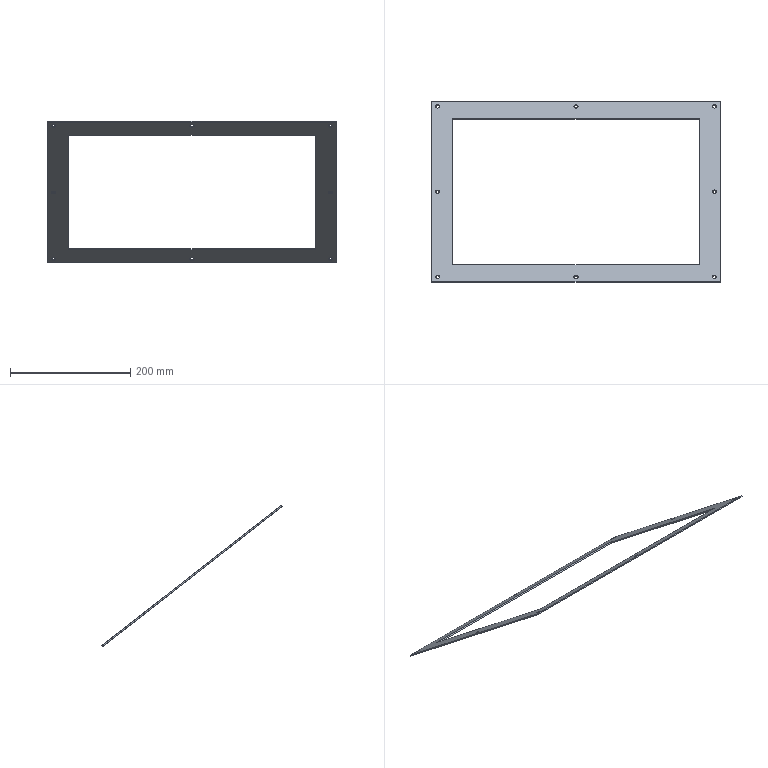Component | SolidWorks | GlassPressFrame-1 | 1 solid | 26 faces | box 480 x 300.68 x 235.53 mm | volume 109996 mm3 | cylinder 16 | plane 10 | commonest cylinder face diameters 7 x14 6.467 x2
build123d program:
from build123d import *

# Parameters (mm, degrees)
SKETCH1_W           = 480
SKETCH1_H           = 380
SKETCH1_W_2         = 410
SKETCH1_H_2         = 310
EXTRUDE_THIN1_DEPTH = 2
SKETCH3_R           = 3.5
SKETCH3_R_2         = 3.233
CUT_EXTRUDE1_DEPTH  = 2


with BuildPart() as part:
    # Sketch1 → Extrude-Thin1 (new body)
    with BuildSketch(Plane.XY):
        with Locations((179.798, -162.283)):
            Rectangle(SKETCH1_W, SKETCH1_H)
        with Locations((179.798, -162.283)):
            Rectangle(SKETCH1_W_2, SKETCH1_H_2, mode=Mode.SUBTRACT)
    extrude(amount=EXTRUDE_THIN1_DEPTH)

    # Sketch3 → Cut-Extrude1 (cut)
    with BuildSketch(Plane(origin=(0, 0, 0), x_dir=(-1, 0, 0), z_dir=(0, 0, -1))):
        with Locations((-409.798, 17.717)):
            Circle(SKETCH3_R)
        with Locations((-179.798, 17.717)):
            Circle(SKETCH3_R)
        with Locations((50.202, 17.717)):
            Circle(SKETCH3_R)
        with Locations((-409.798, -162.283)):
            Circle(SKETCH3_R)
        with Locations((50.202, -162.283)):
            Circle(SKETCH3_R_2)
        with Locations((50.202, -342.283)):
            Circle(SKETCH3_R)
        with Locations((-179.798, -342.283)):
            Circle(SKETCH3_R)
        with Locations((-409.798, -342.283)):
            Circle(SKETCH3_R)
    extrude(amount=-CUT_EXTRUDE1_DEPTH, mode=Mode.SUBTRACT)


solid = part.part

# Placed as in the assembly
solid = solid.moved(Location((-749.348, 310.636, 246.769), (-38, 0, 0)))